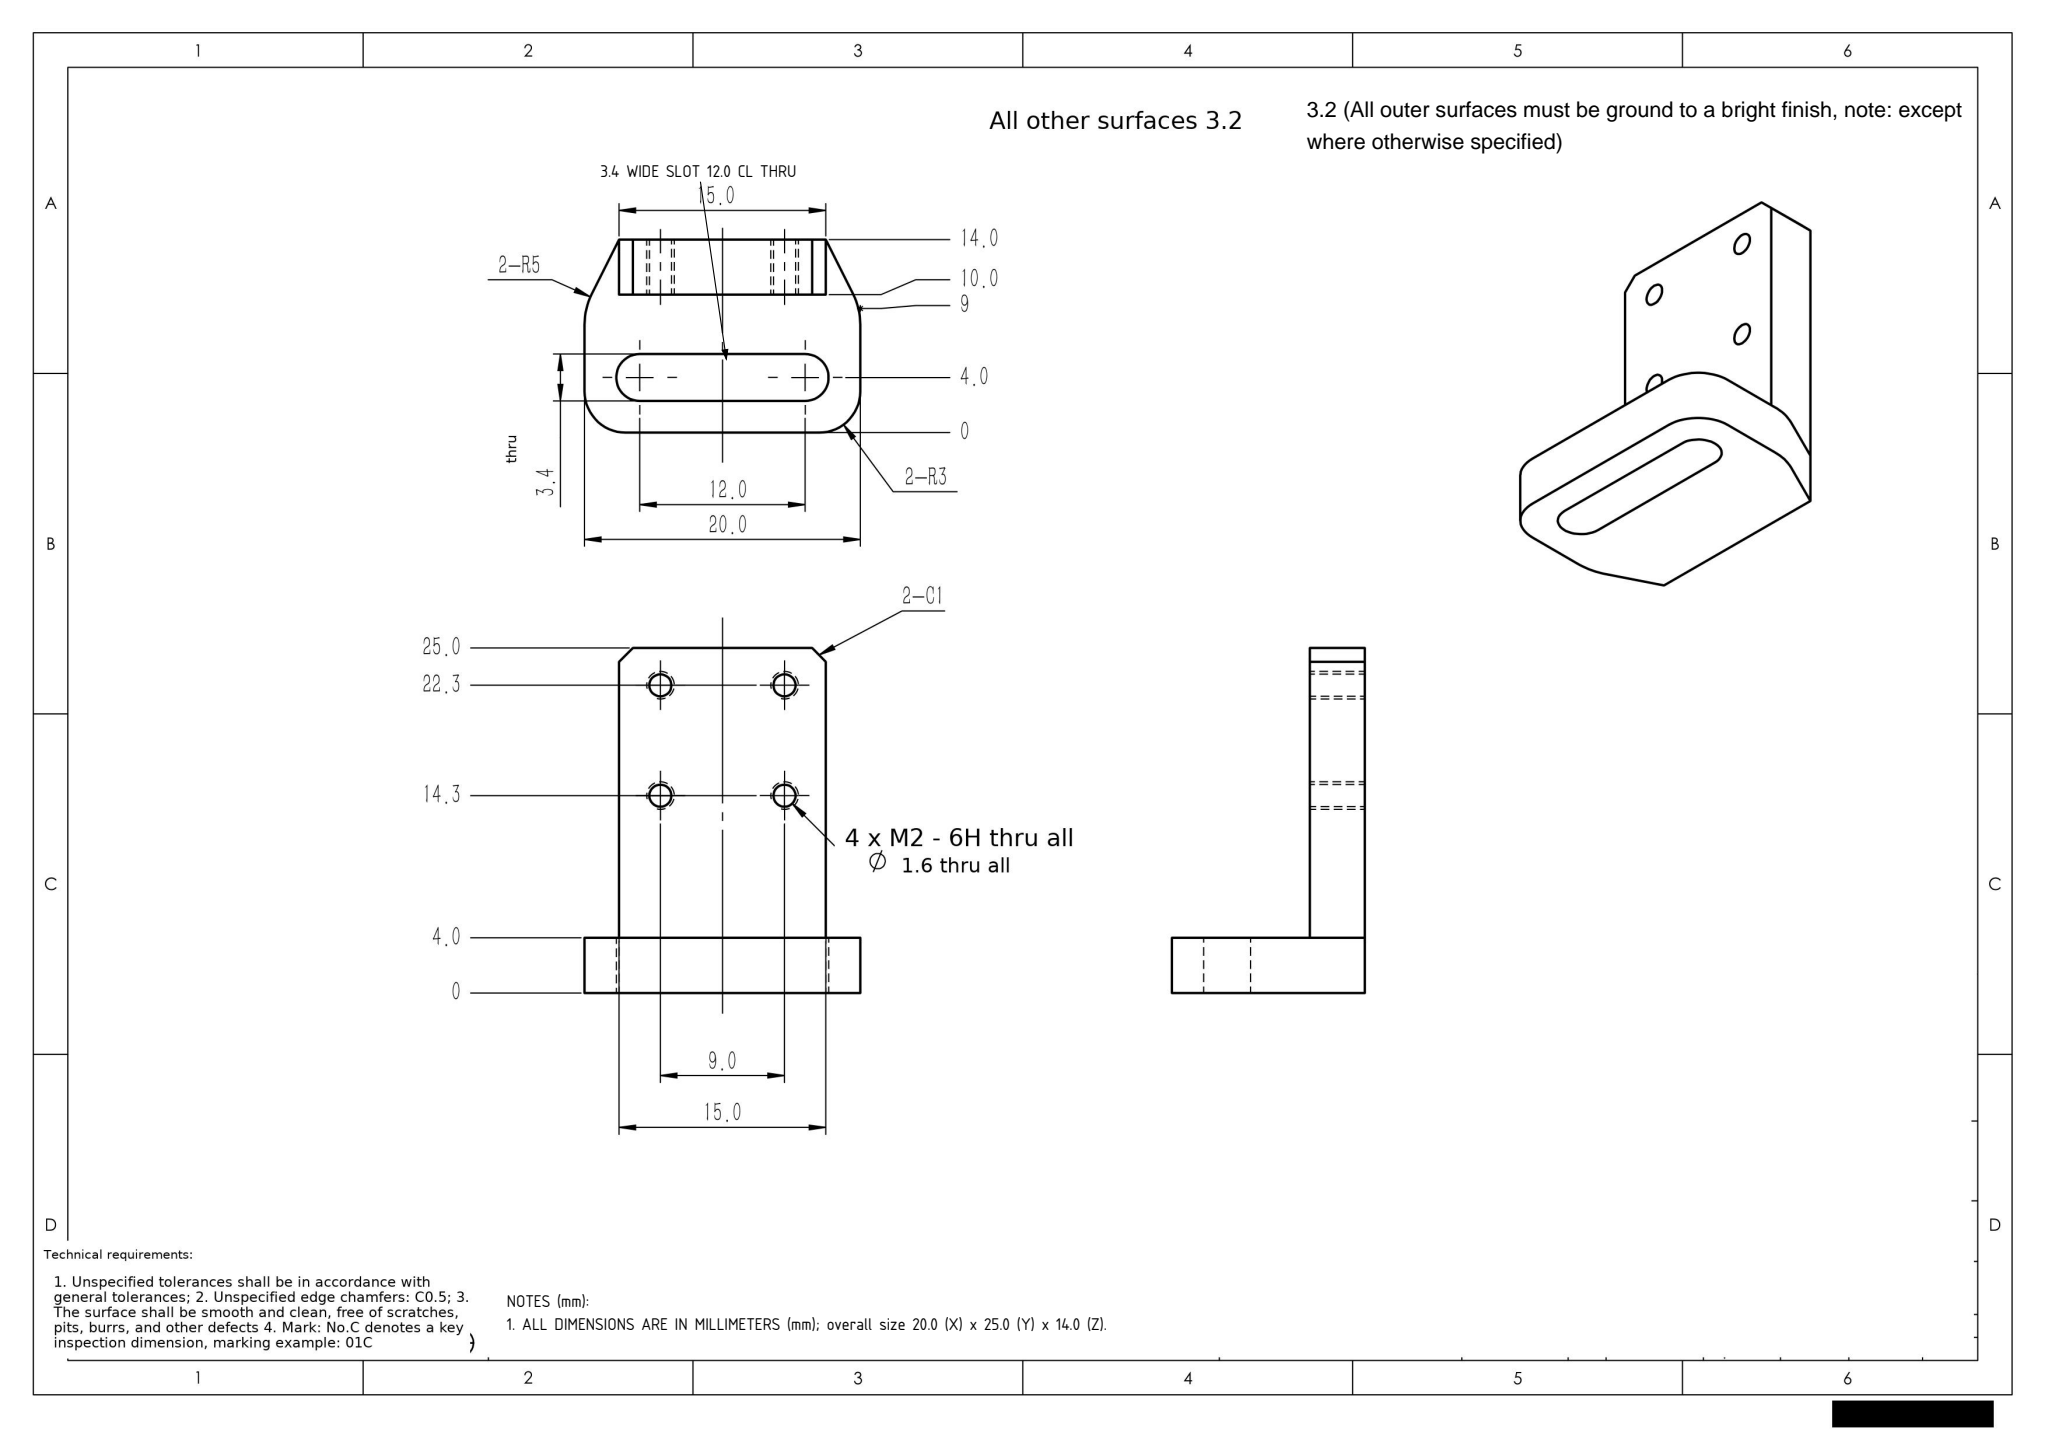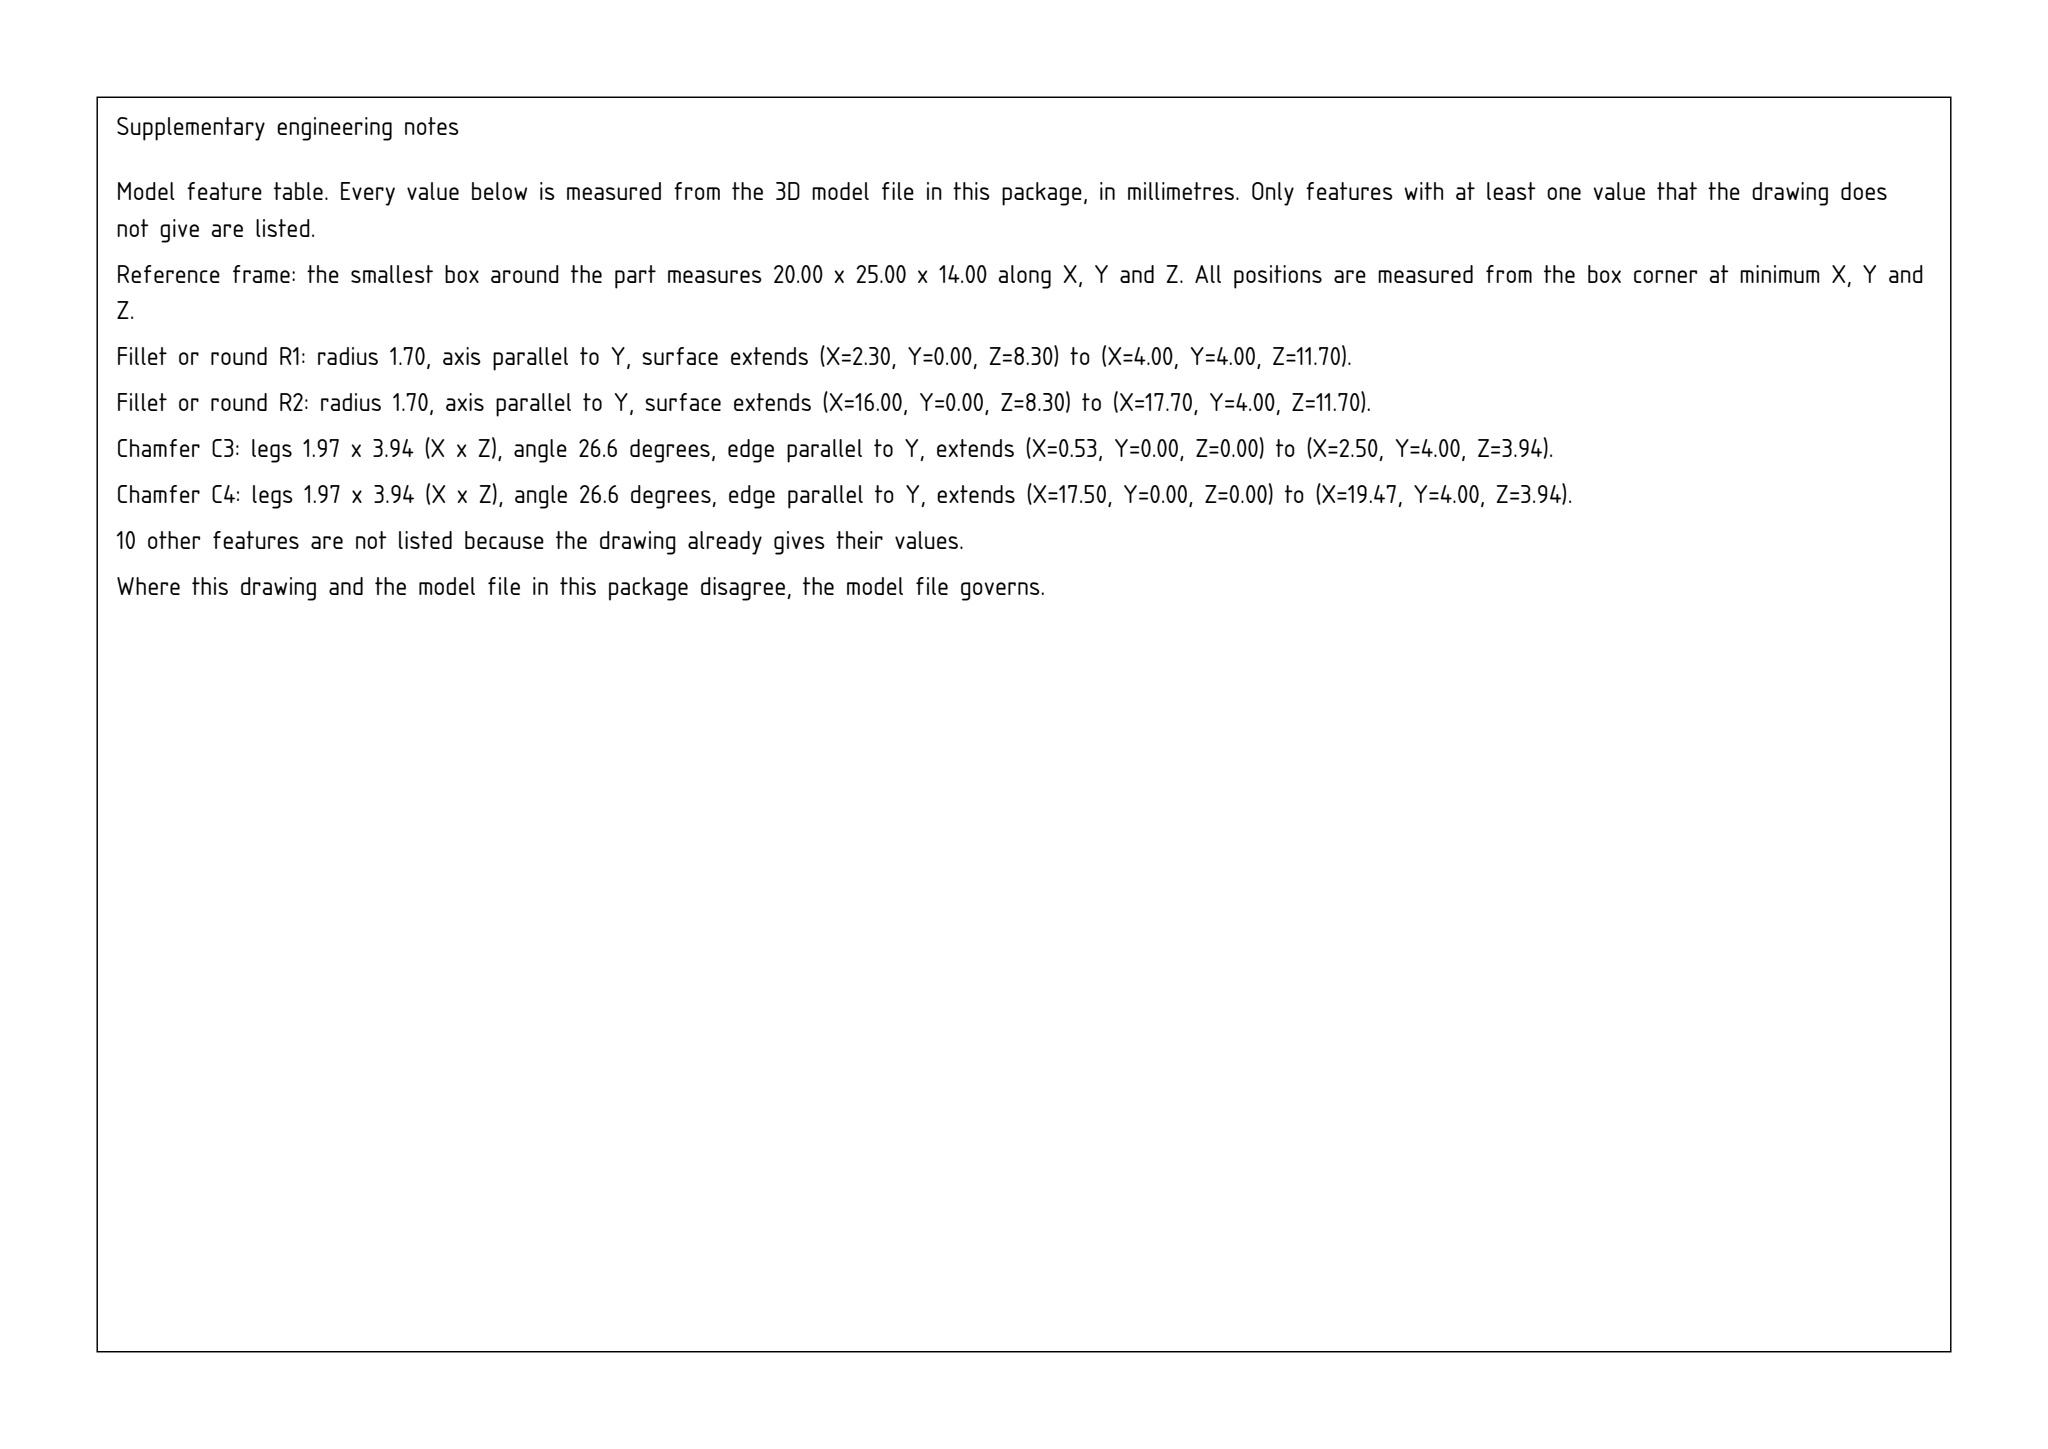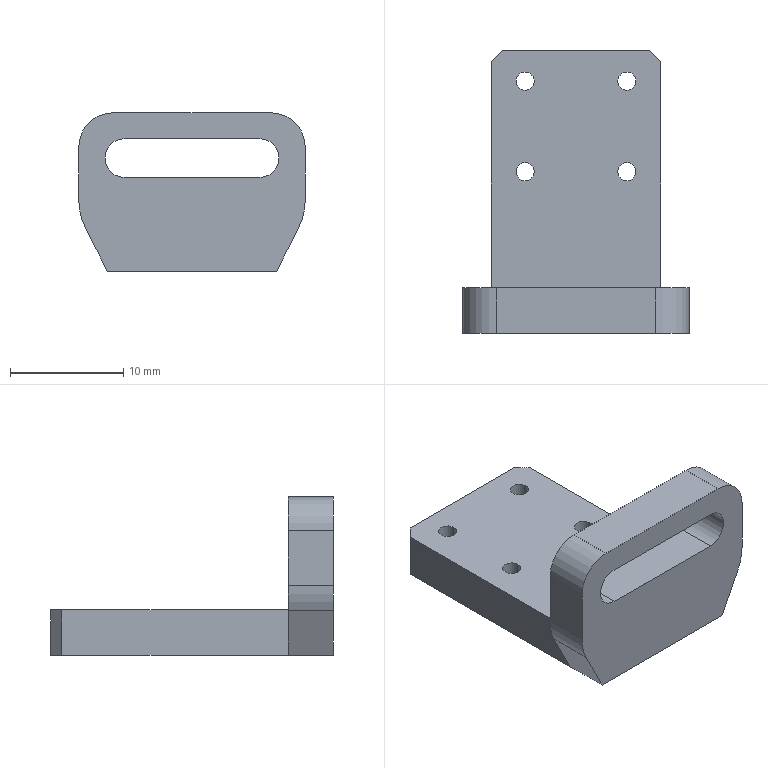Part | SolidWorks | mm | 1 solid | 30 faces | box 20 x 25 x 14 mm | volume 2078 mm3 | plane 16 | cylinder 14 | commonest cylinder face diameters 1.6 x8 3.4 x2 10 x2 6 x2
Drawing notes:
ALL DIMENSIONS ARE IN MILLIMETERS (mm); overall size 20.0 (X) x 25.0 (Y) x 14.0 (Z). | from the solid: STEP model units mm; bbox_xyz [20.0, 25.0, 14.0]
TOP VIEW: SLOT 3.4 WIDE X 12.0 BTWN CL, THRU 4.0 PLATE | from the solid: Ø3.4 cyls, axis Y, at x=4.0 & x=16.0, z=10.0, len 4.0 = full y 0->4.0 plate thickness; CL spacing 16.0-4.0=12.0
build123d program:
from build123d import *

# Parameters (mm, degrees)
SKETCH1_W                  = 20
SKETCH1_H                  = 25
BOSS_EXTRUDE1_DEPTH        = 4
SKETCH2_W                  = 20
SKETCH2_H                  = 4
BOSS_EXTRUDE2_DEPTH        = 10
F_3_4_3_4_DIAMETER_HOLE1_D = 3.4
M2_TAPPED_HOLE1_D          = 1.6
CUT_EXTRUDE1_DEPTH         = 28.148
SKETCH9_W                  = 2.5
SKETCH9_H                  = 21
CUT_EXTRUDE2_DEPTH         = 19.875
CHAMFER1_SIZE              = 2.5
CHAMFER1_SIZE2             = 5
FILLET1_R                  = 5
FILLET2_R                  = 3
CHAMFER3_SIZE              = 1


with BuildPart() as part:
    # Sketch1 → Boss-Extrude1 (new body)
    with BuildSketch(Plane.XY):
        Rectangle(SKETCH1_W, SKETCH1_H)
    extrude(amount=BOSS_EXTRUDE1_DEPTH)

    # Sketch2 → Boss-Extrude2 (add)
    with BuildSketch(Plane.XY.offset(4)):
        with Locations((0, -10.5)):
            Rectangle(SKETCH2_W, SKETCH2_H)
    extrude(amount=BOSS_EXTRUDE2_DEPTH)

    # 3.4 _3.4_ Diameter Hole1 (through all)
    with Locations(Plane(origin=(0, -12.5, 0), x_dir=(-1, 0, 0), z_dir=(0, -1, 0))):
        with Locations((6, -10), (-6, -10)):
            Hole(F_3_4_3_4_DIAMETER_HOLE1_D / 2)

    # M2 Tapped Hole1 (through all)
    with Locations(Plane(origin=(0, 0, 0), x_dir=(-1, 0, 0), z_dir=(0, 0, -1))):
        with Locations((-4.5, 1.8), (-4.5, 9.8), (4.5, 9.8), (4.5, 1.8)):
            Hole(M2_TAPPED_HOLE1_D / 2)

    # Sketch8 → Cut-Extrude1 (cut, through all)
    with BuildSketch(Plane(origin=(0, -8.5, 0), x_dir=(1, 0, 0), z_dir=(0, 1, 0))):
        with BuildLine():
            Line((-6, -8.3), (6, -8.3))
            ThreePointArc((6, -8.3), (7.7, -10), (6, -11.7))
            Line((6, -11.7), (-6, -11.7))
            ThreePointArc((-6, -11.7), (-7.7, -10), (-6, -8.3))
        make_face()
    extrude(amount=-CUT_EXTRUDE1_DEPTH, mode=Mode.SUBTRACT)

    # Sketch9 → Cut-Extrude2 (cut, through all)
    with BuildSketch(Plane.XY.offset(4)):
        with Locations((8.75, 2)):
            Rectangle(SKETCH9_W, SKETCH9_H)
        with Locations((-8.75, 2)):
            Rectangle(SKETCH9_W, SKETCH9_H)
    extrude(amount=-CUT_EXTRUDE2_DEPTH, mode=Mode.SUBTRACT)

    # Chamfer1
    chamfer1_edges = [part.edges().sort_by_distance(p)[0] for p in [
        (-10, -10.5, 0),
        (10, -10.5, 0),
    ]]
    chamfer1_side = [part.faces().sort_by_distance(p)[0] for p in [
        (0, -0.6632, 0),
    ]]
    chamfer(chamfer1_edges, length=CHAMFER1_SIZE, length2=CHAMFER1_SIZE2, reference=chamfer1_side[0])

    # Fillet1
    fillet1_edges = [part.edges().sort_by_distance(p)[0] for p in [
        (-10, -10.5, 5),
        (10, -10.5, 5),
    ]]
    fillet(fillet1_edges, radius=FILLET1_R)

    # Fillet2
    fillet2_edges = [part.edges().sort_by_distance(p)[0] for p in [
        (-10, -10.5, 14),
        (10, -10.5, 14),
    ]]
    fillet(fillet2_edges, radius=FILLET2_R)

    # Chamfer3
    chamfer3_edges = [part.edges().sort_by_distance(p)[0] for p in [
        (7.5, 12.5, 2),
        (-7.5, 12.5, 2),
    ]]
    chamfer(chamfer3_edges, length=CHAMFER3_SIZE)


solid = part.part